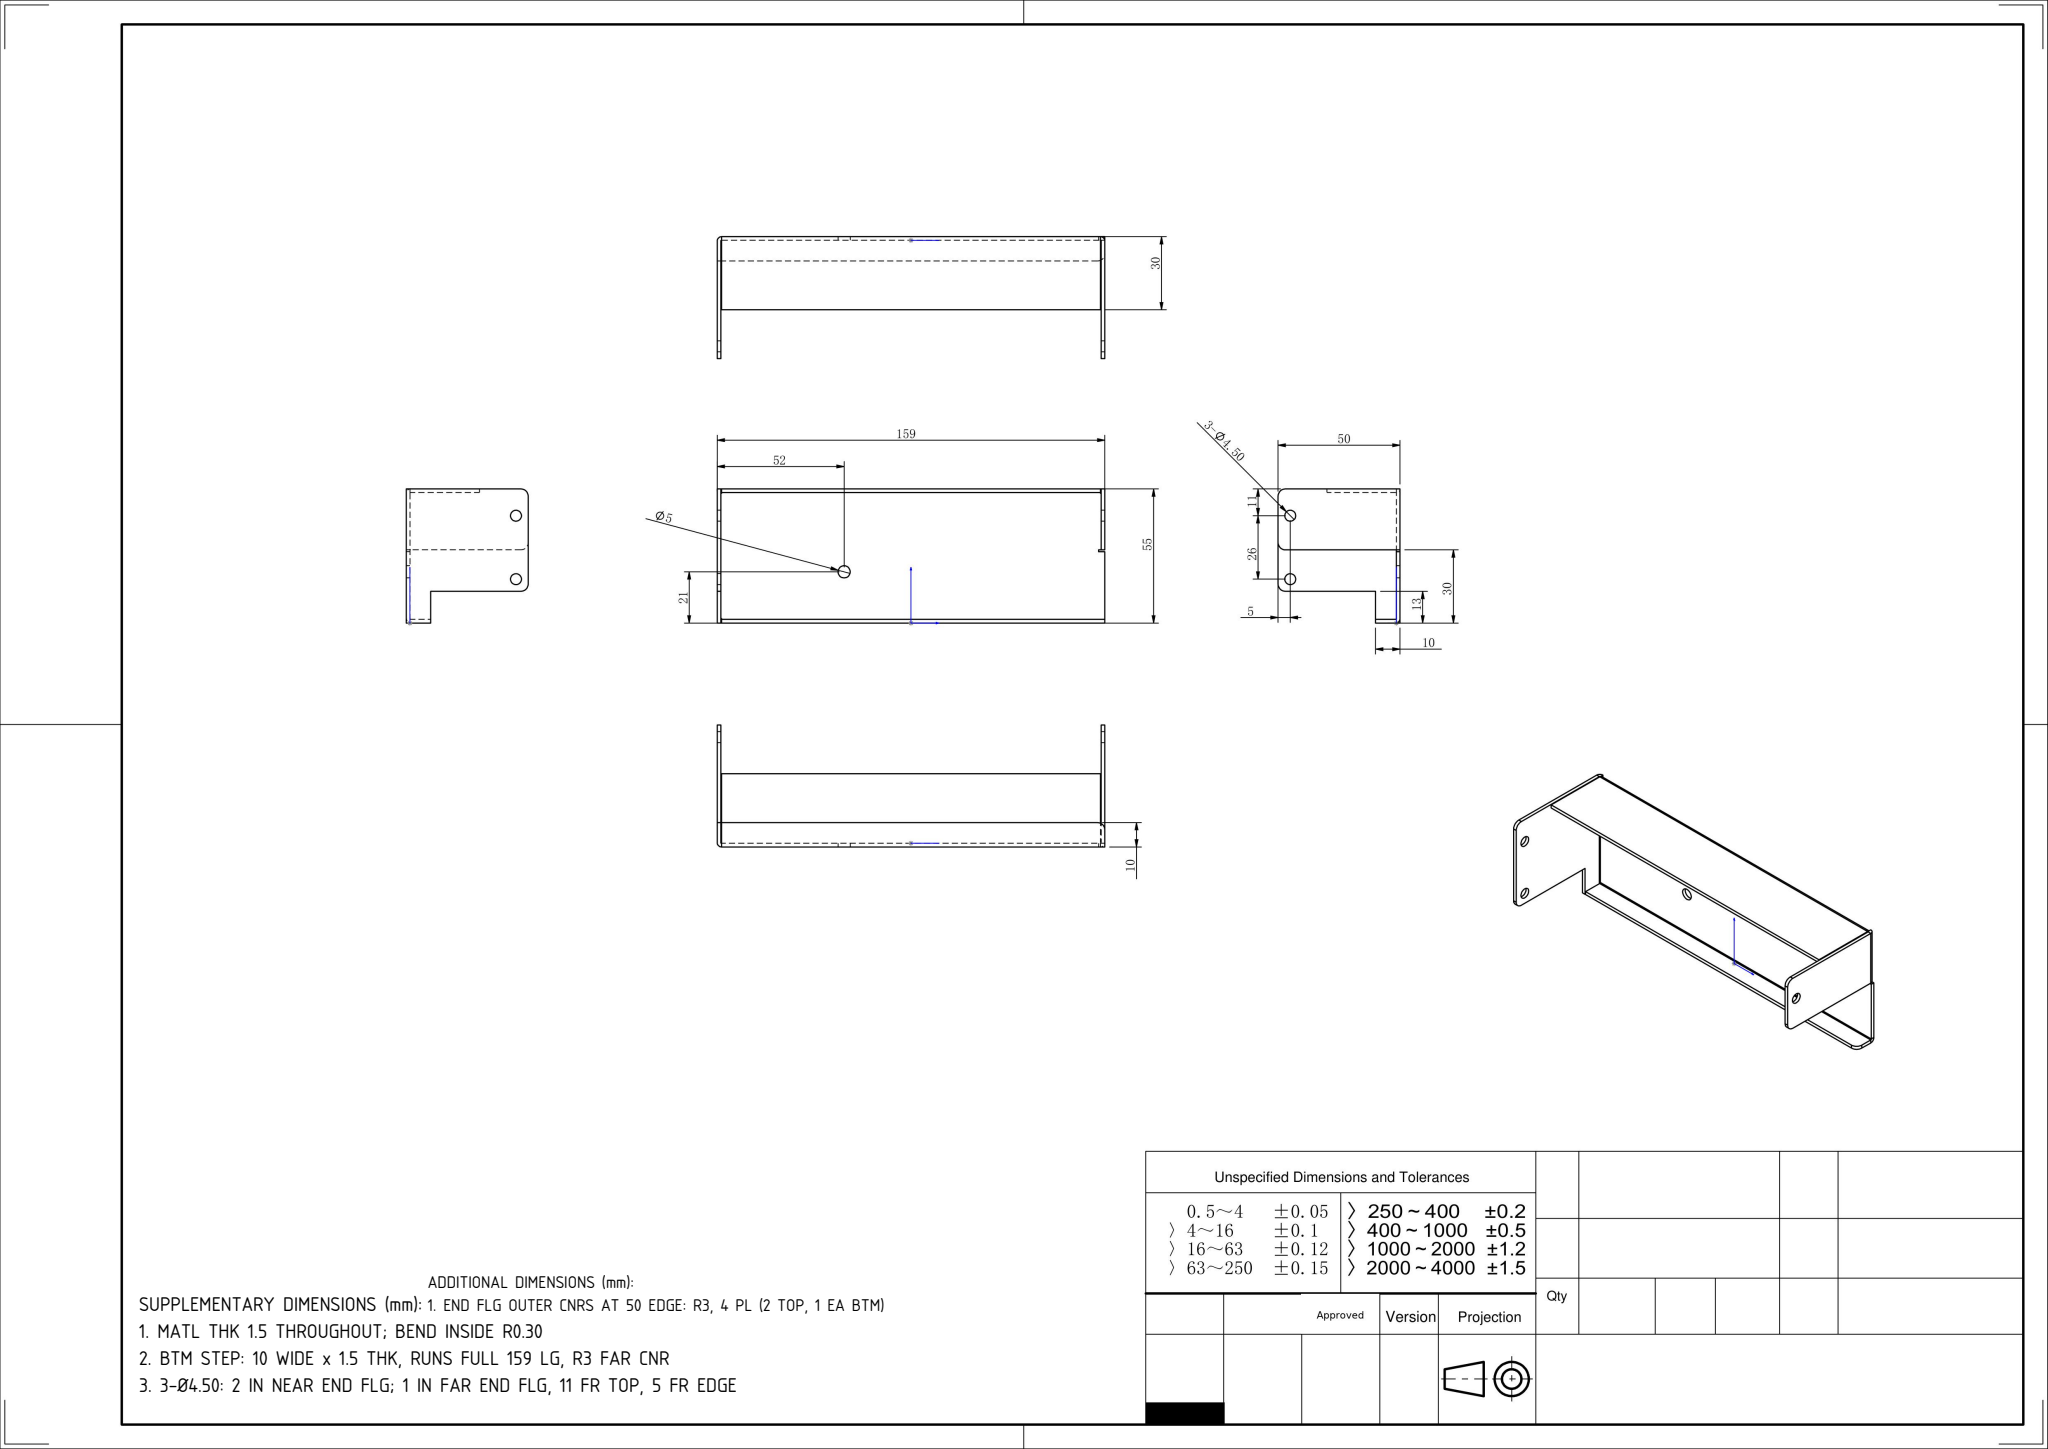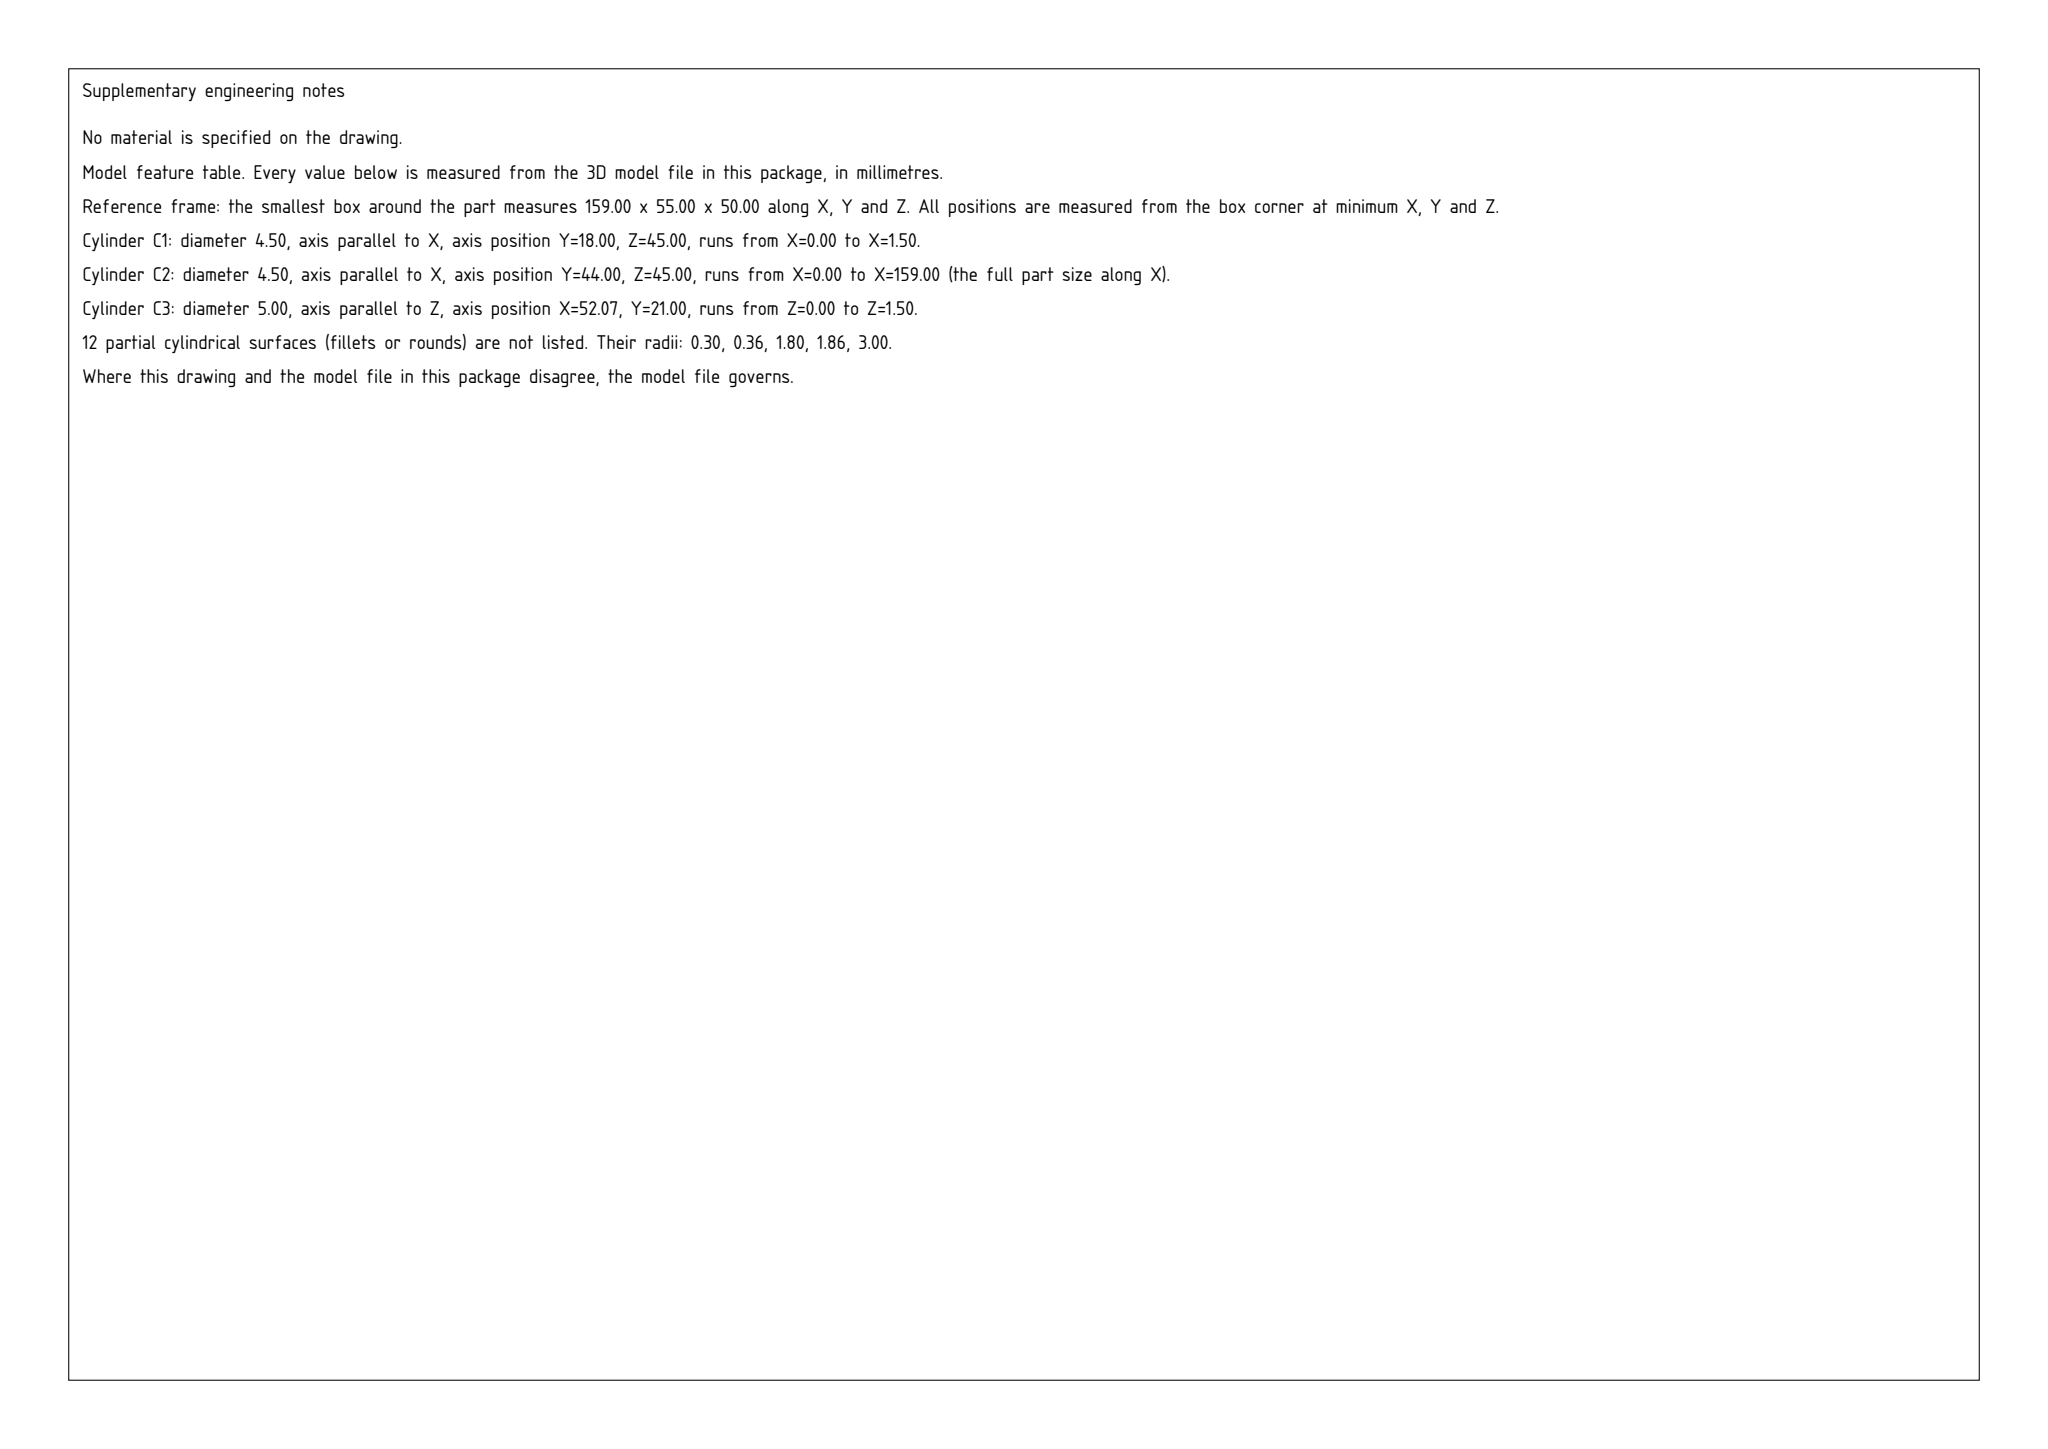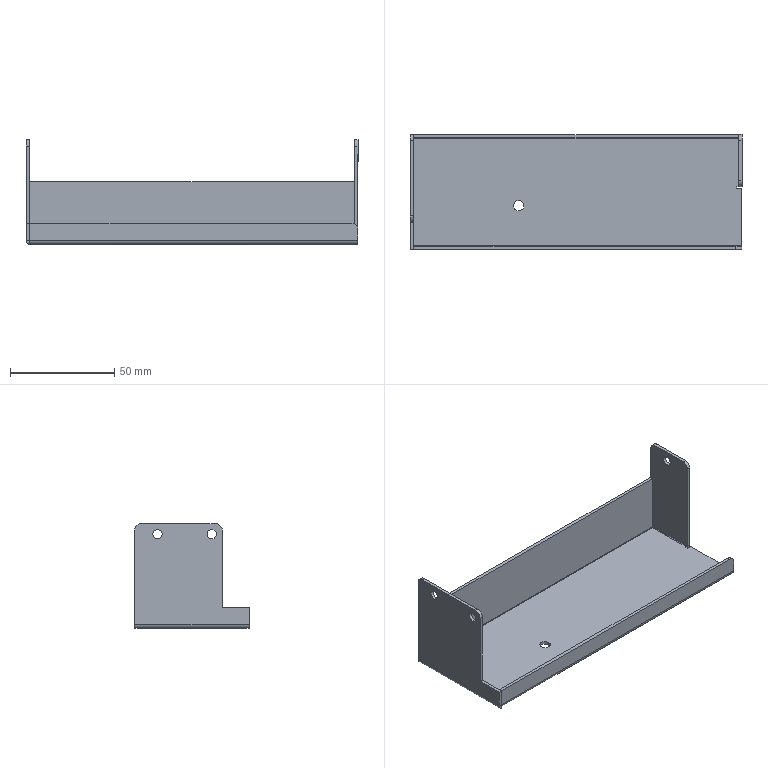Part | SolidWorks | mm | 1 solid | 60 faces | box 159 x 55 x 50 mm | volume 26415 mm3 | plane 39 | cylinder 21 | commonest cylinder face diameters 4.5 x6 6 x5 3.6 x3 0.6 x3 5 x2 3.72 x1 0.72 x1